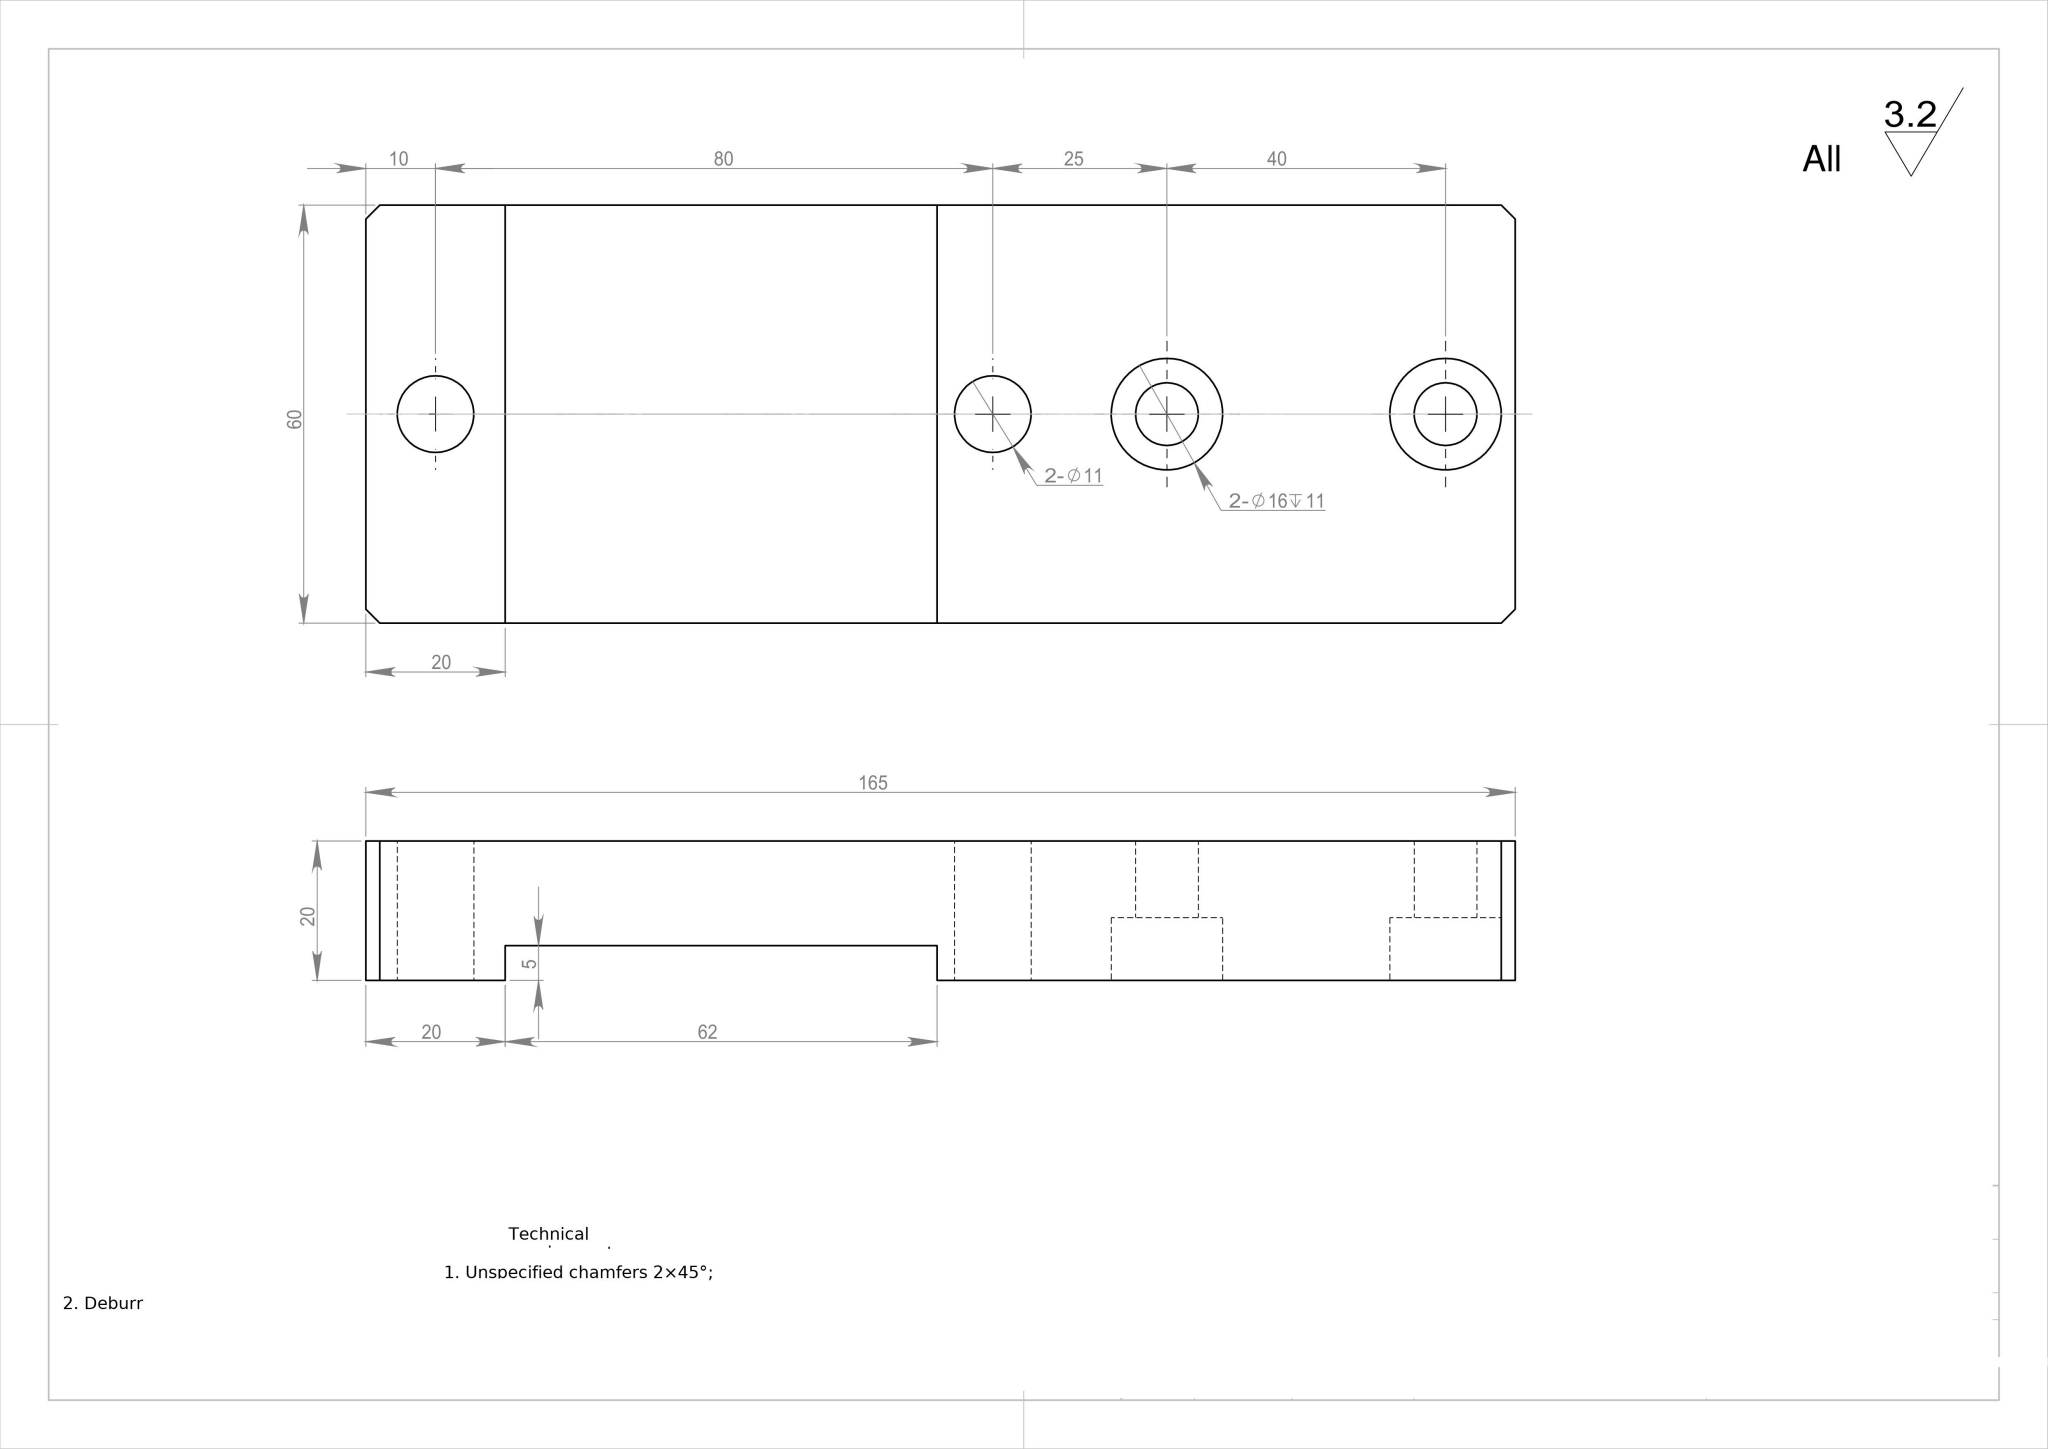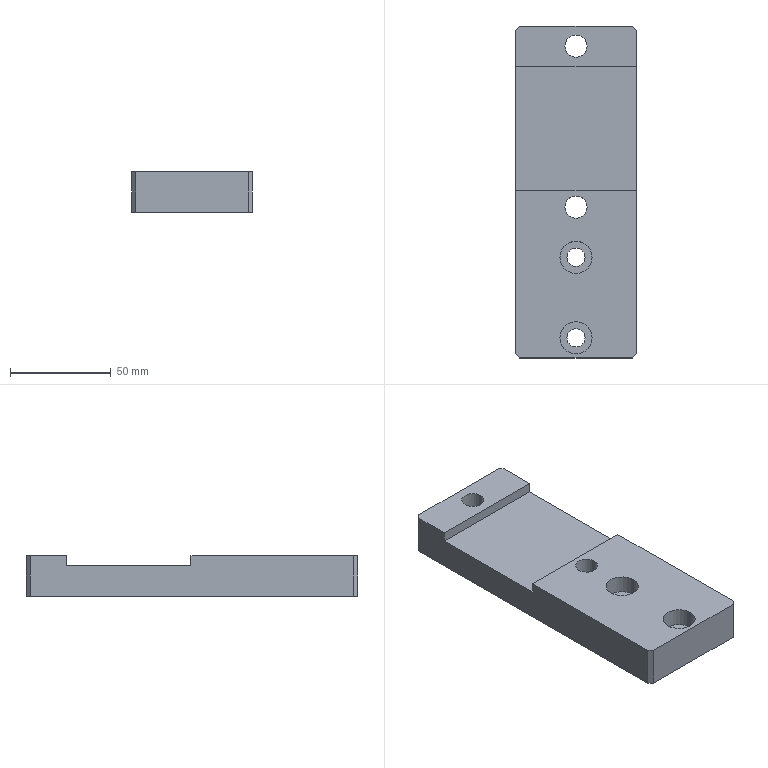Part | SolidWorks | mm | 1 solid | 28 faces | box 60 x 165 x 20 mm | volume 170420 mm3 | plane 16 | cylinder 12 | commonest cylinder face diameters 16 x4 9 x4 11 x4
build123d program:
from build123d import *

# Parameters (mm, degrees)
SKETCH1_W                                         = 60
SKETCH1_H                                         = 165
BOSS_EXTRUDE1_DEPTH                               = 20
SKETCH2_R                                         = 5.5
CUT_EXTRUDE1_DEPTH                                = 91.035
LPATTERN1_COUNT                                   = 2
LPATTERN1_PITCH                                   = 80
SKETCH3_W                                         = 60
SKETCH3_H                                         = 62
CUT_EXTRUDE2_DEPTH                                = 5
HOLE_SIZE_ACCORDING_TO_TYPE_1_OF_HEXA_D           = 9
HOLE_SIZE_ACCORDING_TO_TYPE_1_OF_HEXA_CBORE_D     = 16
HOLE_SIZE_ACCORDING_TO_TYPE_1_OF_HEXA_CBORE_DEPTH = 9
CHAMFER1_SIZE                                     = 2


with BuildPart() as part:
    # Sketch1 → Boss-Extrude1 (new body)
    with BuildSketch(Plane.XY):
        Rectangle(SKETCH1_W, SKETCH1_H)
    extrude(amount=BOSS_EXTRUDE1_DEPTH)

    # Sketch2 → Cut-Extrude1 (cut, through all)
    with BuildSketch(Plane(origin=(0, 0, 0), x_dir=(-1, 0, 0), z_dir=(0, 0, -1))):
        with Locations((0, 72.5)):
            Circle(SKETCH2_R)
    cut_extrude1 = extrude(amount=-CUT_EXTRUDE1_DEPTH, mode=Mode.SUBTRACT)

    # LPattern1: Cut-Extrude1 ×2
    with Locations(*[(0, -i * LPATTERN1_PITCH, 0) for i in range(1, LPATTERN1_COUNT)]):
        add(cut_extrude1, mode=Mode.SUBTRACT)

    # Sketch3 → Cut-Extrude2 (cut)
    with BuildSketch(Plane(origin=(0, 0, 20), x_dir=(-1, 0, 0), z_dir=(0, 0, -1))):
        with Locations((0, 31.5)):
            Rectangle(SKETCH3_W, SKETCH3_H)
    extrude(amount=CUT_EXTRUDE2_DEPTH, mode=Mode.SUBTRACT)

    # Hole Size _ according to_ Type 1 of Hexa (through all)
    with Locations(Plane.XY.offset(20)):
        with Locations((0, -32.5), (0, -72.5)):
            CounterBoreHole(HOLE_SIZE_ACCORDING_TO_TYPE_1_OF_HEXA_D / 2, HOLE_SIZE_ACCORDING_TO_TYPE_1_OF_HEXA_CBORE_D / 2, HOLE_SIZE_ACCORDING_TO_TYPE_1_OF_HEXA_CBORE_DEPTH)

    # Chamfer1
    chamfer1_edges = [part.edges().sort_by_distance(p)[0] for p in [
        (30, -82.5, 10),
        (-30, -82.5, 10),
        (-30, 82.5, 10),
        (30, 82.5, 10),
    ]]
    chamfer(chamfer1_edges, length=CHAMFER1_SIZE)


solid = part.part
STEP:
#1=CARTESIAN_POINT('',(-8.,-32.5,11.));
#2=VERTEX_POINT('',#1);
#3=CARTESIAN_POINT('',(8.,-32.5,11.));
#4=VERTEX_POINT('',#3);
#5=CARTESIAN_POINT('',(-0.,-32.5,11.));
#6=DIRECTION('',(0.,0.,1.));
#7=DIRECTION('',(1.,0.,0.));
#8=AXIS2_PLACEMENT_3D('',#5,#6,#7);
#9=CIRCLE('',#8,8.);
#10=EDGE_CURVE('',#2,#4,#9,.T.);
#11=ORIENTED_EDGE('',*,*,#10,.F.);
#12=CARTESIAN_POINT('',(-8.,-32.5,20.));
#13=VERTEX_POINT('',#12);
#14=CARTESIAN_POINT('',(-8.,-32.5,20.));
#15=DIRECTION('',(0.,0.,1.));
#16=VECTOR('',#15,1000.);
#17=LINE('',#14,#16);
#18=EDGE_CURVE('',#2,#13,#17,.T.);
#19=ORIENTED_EDGE('',*,*,#18,.T.);
#20=CARTESIAN_POINT('',(8.,-32.5,20.));
#21=VERTEX_POINT('',#20);
#22=CARTESIAN_POINT('',(-0.,-32.5,20.));
#23=DIRECTION('',(0.,0.,1.));
#24=DIRECTION('',(1.,0.,0.));
#25=AXIS2_PLACEMENT_3D('',#22,#23,#24);
#26=CIRCLE('',#25,8.);
#27=EDGE_CURVE('',#13,#21,#26,.T.);
#28=ORIENTED_EDGE('',*,*,#27,.T.);
#29=CARTESIAN_POINT('',(8.,-32.5,20.));
#30=DIRECTION('',(0.,0.,1.));
#31=VECTOR('',#30,1000.);
#32=LINE('',#29,#31);
#33=EDGE_CURVE('',#4,#21,#32,.T.);
#34=ORIENTED_EDGE('',*,*,#33,.F.);
#35=EDGE_LOOP('',(#11,#19,#28,#34));
#36=FACE_OUTER_BOUND('',#35,.T.);
#37=CARTESIAN_POINT('',(-0.,-32.5,20.));
#38=DIRECTION('',(0.,0.,1.));
#39=DIRECTION('',(1.,0.,0.));
#40=AXIS2_PLACEMENT_3D('',#37,#38,#39);
#41=CYLINDRICAL_SURFACE('',#40,8.);
#42=ADVANCED_FACE('',(#36),#41,.F.);
#43=CARTESIAN_POINT('',(-4.5,-32.5,0.));
#44=VERTEX_POINT('',#43);
#45=CARTESIAN_POINT('',(4.5,-32.5,0.));
#46=VERTEX_POINT('',#45);
#47=CARTESIAN_POINT('',(-0.,-32.5,0.));
#48=DIRECTION('',(0.,0.,1.));
#49=DIRECTION('',(1.,0.,0.));
#50=AXIS2_PLACEMENT_3D('',#47,#48,#49);
#51=CIRCLE('',#50,4.5);
#52=EDGE_CURVE('',#44,#46,#51,.T.);
#53=ORIENTED_EDGE('',*,*,#52,.F.);
#54=CARTESIAN_POINT('',(-4.5,-32.5,11.));
#55=VERTEX_POINT('',#54);
#56=CARTESIAN_POINT('',(-4.5,-32.5,20.));
#57=DIRECTION('',(0.,0.,1.));
#58=VECTOR('',#57,1000.);
#59=LINE('',#56,#58);
#60=EDGE_CURVE('',#44,#55,#59,.T.);
#61=ORIENTED_EDGE('',*,*,#60,.T.);
#62=CARTESIAN_POINT('',(4.5,-32.5,11.));
#63=VERTEX_POINT('',#62);
#64=CARTESIAN_POINT('',(-0.,-32.5,11.));
#65=DIRECTION('',(0.,0.,1.));
#66=DIRECTION('',(1.,0.,0.));
#67=AXIS2_PLACEMENT_3D('',#64,#65,#66);
#68=CIRCLE('',#67,4.5);
#69=EDGE_CURVE('',#55,#63,#68,.T.);
#70=ORIENTED_EDGE('',*,*,#69,.T.);
#71=CARTESIAN_POINT('',(4.5,-32.5,20.));
#72=DIRECTION('',(0.,0.,1.));
#73=VECTOR('',#72,1000.);
#74=LINE('',#71,#73);
#75=EDGE_CURVE('',#46,#63,#74,.T.);
#76=ORIENTED_EDGE('',*,*,#75,.F.);
#77=EDGE_LOOP('',(#53,#61,#70,#76));
#78=FACE_OUTER_BOUND('',#77,.T.);
#79=CARTESIAN_POINT('',(-0.,-32.5,20.));
#80=DIRECTION('',(0.,0.,1.));
#81=DIRECTION('',(1.,0.,0.));
#82=AXIS2_PLACEMENT_3D('',#79,#80,#81);
#83=CYLINDRICAL_SURFACE('',#82,4.5);
#84=ADVANCED_FACE('',(#78),#83,.F.);
#85=CARTESIAN_POINT('',(-8.,-72.5,11.));
#86=VERTEX_POINT('',#85);
#87=CARTESIAN_POINT('',(8.,-72.5,11.));
#88=VERTEX_POINT('',#87);
#89=CARTESIAN_POINT('',(-0.,-72.5,11.));
#90=DIRECTION('',(0.,0.,1.));
#91=DIRECTION('',(1.,0.,0.));
#92=AXIS2_PLACEMENT_3D('',#89,#90,#91);
#93=CIRCLE('',#92,8.);
#94=EDGE_CURVE('',#86,#88,#93,.T.);
#95=ORIENTED_EDGE('',*,*,#94,.F.);
#96=CARTESIAN_POINT('',(-8.,-72.5,20.));
#97=VERTEX_POINT('',#96);
#98=CARTESIAN_POINT('',(-8.,-72.5,20.));
#99=DIRECTION('',(0.,0.,1.));
#100=VECTOR('',#99,1000.);
#101=LINE('',#98,#100);
#102=EDGE_CURVE('',#86,#97,#101,.T.);
#103=ORIENTED_EDGE('',*,*,#102,.T.);
#104=CARTESIAN_POINT('',(8.,-72.5,20.));
#105=VERTEX_POINT('',#104);
#106=CARTESIAN_POINT('',(-0.,-72.5,20.));
#107=DIRECTION('',(0.,0.,1.));
#108=DIRECTION('',(1.,0.,0.));
#109=AXIS2_PLACEMENT_3D('',#106,#107,#108);
#110=CIRCLE('',#109,8.);
#111=EDGE_CURVE('',#97,#105,#110,.T.);
#112=ORIENTED_EDGE('',*,*,#111,.T.);
#113=CARTESIAN_POINT('',(8.,-72.5,20.));
#114=DIRECTION('',(0.,0.,1.));
#115=VECTOR('',#114,1000.);
#116=LINE('',#113,#115);
#117=EDGE_CURVE('',#88,#105,#116,.T.);
#118=ORIENTED_EDGE('',*,*,#117,.F.);
#119=EDGE_LOOP('',(#95,#103,#112,#118));
#120=FACE_OUTER_BOUND('',#119,.T.);
#121=CARTESIAN_POINT('',(-0.,-72.5,20.));
#122=DIRECTION('',(0.,0.,1.));
#123=DIRECTION('',(1.,0.,0.));
#124=AXIS2_PLACEMENT_3D('',#121,#122,#123);
#125=CYLINDRICAL_SURFACE('',#124,8.);
#126=ADVANCED_FACE('',(#120),#125,.F.);
#127=CARTESIAN_POINT('',(-4.5,-72.5,0.));
#128=VERTEX_POINT('',#127);
#129=CARTESIAN_POINT('',(4.5,-72.5,0.));
#130=VERTEX_POINT('',#129);
#131=CARTESIAN_POINT('',(-0.,-72.5,0.));
#132=DIRECTION('',(0.,0.,1.));
#133=DIRECTION('',(1.,0.,0.));
#134=AXIS2_PLACEMENT_3D('',#131,#132,#133);
#135=CIRCLE('',#134,4.5);
#136=EDGE_CURVE('',#128,#130,#135,.T.);
#137=ORIENTED_EDGE('',*,*,#136,.F.);
#138=CARTESIAN_POINT('',(-4.5,-72.5,11.));
#139=VERTEX_POINT('',#138);
#140=CARTESIAN_POINT('',(-4.5,-72.5,20.));
#141=DIRECTION('',(0.,0.,1.));
#142=VECTOR('',#141,1000.);
#143=LINE('',#140,#142);
#144=EDGE_CURVE('',#128,#139,#143,.T.);
#145=ORIENTED_EDGE('',*,*,#144,.T.);
#146=CARTESIAN_POINT('',(4.5,-72.5,11.));
#147=VERTEX_POINT('',#146);
#148=CARTESIAN_POINT('',(-0.,-72.5,11.));
#149=DIRECTION('',(0.,0.,1.));
#150=DIRECTION('',(1.,0.,0.));
#151=AXIS2_PLACEMENT_3D('',#148,#149,#150);
#152=CIRCLE('',#151,4.5);
#153=EDGE_CURVE('',#139,#147,#152,.T.);
#154=ORIENTED_EDGE('',*,*,#153,.T.);
#155=CARTESIAN_POINT('',(4.5,-72.5,20.));
#156=DIRECTION('',(0.,0.,1.));
#157=VECTOR('',#156,1000.);
#158=LINE('',#155,#157);
#159=EDGE_CURVE('',#130,#147,#158,.T.);
#160=ORIENTED_EDGE('',*,*,#159,.F.);
#161=EDGE_LOOP('',(#137,#145,#154,#160));
#162=FACE_OUTER_BOUND('',#161,.T.);
#163=CARTESIAN_POINT('',(-0.,-72.5,20.));
#164=DIRECTION('',(0.,0.,1.));
#165=DIRECTION('',(1.,0.,0.));
#166=AXIS2_PLACEMENT_3D('',#163,#164,#165);
#167=CYLINDRICAL_SURFACE('',#166,4.5);
#168=ADVANCED_FACE('',(#162),#167,.F.);
#169=CARTESIAN_POINT('',(5.5,-7.5,20.));
#170=VERTEX_POINT('',#169);
#171=CARTESIAN_POINT('',(-5.5,-7.5,20.));
#172=VERTEX_POINT('',#171);
#173=CARTESIAN_POINT('',(0.,-7.5,20.));
#174=DIRECTION('',(0.,0.,-1.));
#175=DIRECTION('',(-1.,0.,0.));
#176=AXIS2_PLACEMENT_3D('',#173,#174,#175);
#177=CIRCLE('',#176,5.5);
#178=EDGE_CURVE('',#170,#172,#177,.T.);
#179=ORIENTED_EDGE('',*,*,#178,.F.);
#180=CARTESIAN_POINT('',(5.5,-7.5,0.));
#181=VERTEX_POINT('',#180);
#182=CARTESIAN_POINT('',(5.5,-7.5,20.));
#183=DIRECTION('',(0.,0.,-1.));
#184=VECTOR('',#183,1000.);
#185=LINE('',#182,#184);
#186=EDGE_CURVE('',#170,#181,#185,.T.);
#187=ORIENTED_EDGE('',*,*,#186,.T.);
#188=CARTESIAN_POINT('',(-5.5,-7.5,0.));
#189=VERTEX_POINT('',#188);
#190=CARTESIAN_POINT('',(0.,-7.5,0.));
#191=DIRECTION('',(0.,0.,-1.));
#192=DIRECTION('',(-1.,0.,0.));
#193=AXIS2_PLACEMENT_3D('',#190,#191,#192);
#194=CIRCLE('',#193,5.5);
#195=EDGE_CURVE('',#181,#189,#194,.T.);
#196=ORIENTED_EDGE('',*,*,#195,.T.);
#197=CARTESIAN_POINT('',(-5.5,-7.5,20.));
#198=DIRECTION('',(0.,0.,-1.));
#199=VECTOR('',#198,1000.);
#200=LINE('',#197,#199);
#201=EDGE_CURVE('',#172,#189,#200,.T.);
#202=ORIENTED_EDGE('',*,*,#201,.F.);
#203=EDGE_LOOP('',(#179,#187,#196,#202));
#204=FACE_OUTER_BOUND('',#203,.T.);
#205=CARTESIAN_POINT('',(0.,-7.5,20.));
#206=DIRECTION('',(0.,0.,-1.));
#207=DIRECTION('',(-1.,0.,0.));
#208=AXIS2_PLACEMENT_3D('',#205,#206,#207);
#209=CYLINDRICAL_SURFACE('',#208,5.5);
#210=ADVANCED_FACE('',(#204),#209,.F.);
#211=CARTESIAN_POINT('',(5.5,72.5,20.));
#212=VERTEX_POINT('',#211);
#213=CARTESIAN_POINT('',(-5.5,72.5,20.));
#214=VERTEX_POINT('',#213);
#215=CARTESIAN_POINT('',(0.,72.5,20.));
#216=DIRECTION('',(0.,0.,-1.));
#217=DIRECTION('',(-1.,0.,0.));
#218=AXIS2_PLACEMENT_3D('',#215,#216,#217);
#219=CIRCLE('',#218,5.5);
#220=EDGE_CURVE('',#212,#214,#219,.T.);
#221=ORIENTED_EDGE('',*,*,#220,.F.);
#222=CARTESIAN_POINT('',(5.5,72.5,0.));
#223=VERTEX_POINT('',#222);
#224=CARTESIAN_POINT('',(5.5,72.5,20.));
#225=DIRECTION('',(0.,0.,-1.));
#226=VECTOR('',#225,1000.);
#227=LINE('',#224,#226);
#228=EDGE_CURVE('',#212,#223,#227,.T.);
#229=ORIENTED_EDGE('',*,*,#228,.T.);
#230=CARTESIAN_POINT('',(-5.5,72.5,0.));
#231=VERTEX_POINT('',#230);
#232=CARTESIAN_POINT('',(0.,72.5,0.));
#233=DIRECTION('',(0.,0.,-1.));
#234=DIRECTION('',(-1.,0.,0.));
#235=AXIS2_PLACEMENT_3D('',#232,#233,#234);
#236=CIRCLE('',#235,5.5);
#237=EDGE_CURVE('',#223,#231,#236,.T.);
#238=ORIENTED_EDGE('',*,*,#237,.T.);
#239=CARTESIAN_POINT('',(-5.5,72.5,20.));
#240=DIRECTION('',(0.,0.,-1.));
#241=VECTOR('',#240,1000.);
#242=LINE('',#239,#241);
#243=EDGE_CURVE('',#214,#231,#242,.T.);
#244=ORIENTED_EDGE('',*,*,#243,.F.);
#245=EDGE_LOOP('',(#221,#229,#238,#244));
#246=FACE_OUTER_BOUND('',#245,.T.);
#247=CARTESIAN_POINT('',(0.,72.5,20.));
#248=DIRECTION('',(0.,0.,-1.));
#249=DIRECTION('',(-1.,0.,0.));
#250=AXIS2_PLACEMENT_3D('',#247,#248,#249);
#251=CYLINDRICAL_SURFACE('',#250,5.5);
#252=ADVANCED_FACE('',(#246),#251,.F.);
#253=CARTESIAN_POINT('',(30.,-80.5,0.));
#254=VERTEX_POINT('',#253);
#255=CARTESIAN_POINT('',(30.,80.5,0.));
#256=VERTEX_POINT('',#255);
#257=CARTESIAN_POINT('',(30.,82.5,0.));
#258=DIRECTION('',(-0.,1.,0.));
#259=VECTOR('',#258,1000.);
#260=LINE('',#257,#259);
#261=EDGE_CURVE('',#254,#256,#260,.T.);
#262=ORIENTED_EDGE('',*,*,#261,.T.);
#263=CARTESIAN_POINT('',(30.,80.5,20.));
#264=VERTEX_POINT('',#263);
#265=CARTESIAN_POINT('',(30.,80.5,20.));
#266=DIRECTION('',(0.,0.,1.));
#267=VECTOR('',#266,1000.);
#268=LINE('',#265,#267);
#269=EDGE_CURVE('',#256,#264,#268,.T.);
#270=ORIENTED_EDGE('',*,*,#269,.T.);
#271=CARTESIAN_POINT('',(30.,62.5,20.));
#272=VERTEX_POINT('',#271);
#273=CARTESIAN_POINT('',(30.,82.5,20.));
#274=DIRECTION('',(-0.,1.,0.));
#275=VECTOR('',#274,1000.);
#276=LINE('',#273,#275);
#277=EDGE_CURVE('',#272,#264,#276,.T.);
#278=ORIENTED_EDGE('',*,*,#277,.F.);
#279=CARTESIAN_POINT('',(30.,62.5,15.));
#280=VERTEX_POINT('',#279);
#281=CARTESIAN_POINT('',(30.,62.5,15.));
#282=DIRECTION('',(0.,0.,1.));
#283=VECTOR('',#282,1000.);
#284=LINE('',#281,#283);
#285=EDGE_CURVE('',#280,#272,#284,.T.);
#286=ORIENTED_EDGE('',*,*,#285,.F.);
#287=CARTESIAN_POINT('',(30.,0.5,15.));
#288=VERTEX_POINT('',#287);
#289=CARTESIAN_POINT('',(30.,62.5,15.));
#290=DIRECTION('',(-0.,-1.,0.));
#291=VECTOR('',#290,1000.);
#292=LINE('',#289,#291);
#293=EDGE_CURVE('',#280,#288,#292,.T.);
#294=ORIENTED_EDGE('',*,*,#293,.T.);
#295=CARTESIAN_POINT('',(30.,0.5,20.));
#296=VERTEX_POINT('',#295);
#297=CARTESIAN_POINT('',(30.,0.5,15.));
#298=DIRECTION('',(0.,0.,1.));
#299=VECTOR('',#298,1000.);
#300=LINE('',#297,#299);
#301=EDGE_CURVE('',#288,#296,#300,.T.);
#302=ORIENTED_EDGE('',*,*,#301,.T.);
#303=CARTESIAN_POINT('',(30.,-80.5,20.));
#304=VERTEX_POINT('',#303);
#305=CARTESIAN_POINT('',(30.,82.5,20.));
#306=DIRECTION('',(-0.,1.,0.));
#307=VECTOR('',#306,1000.);
#308=LINE('',#305,#307);
#309=EDGE_CURVE('',#304,#296,#308,.T.);
#310=ORIENTED_EDGE('',*,*,#309,.F.);
#311=CARTESIAN_POINT('',(30.,-80.5,20.));
#312=DIRECTION('',(0.,0.,-1.));
#313=VECTOR('',#312,1000.);
#314=LINE('',#311,#313);
#315=EDGE_CURVE('',#304,#254,#314,.T.);
#316=ORIENTED_EDGE('',*,*,#315,.T.);
#317=EDGE_LOOP('',(#262,#270,#278,#286,#294,#302,#310,#316));
#318=FACE_OUTER_BOUND('',#317,.T.);
#319=CARTESIAN_POINT('',(30.,82.5,20.));
#320=DIRECTION('',(-1.,-0.,0.));
#321=DIRECTION('',(0.,-1.,0.));
#322=AXIS2_PLACEMENT_3D('',#319,#320,#321);
#323=PLANE('',#322);
#324=ADVANCED_FACE('',(#318),#323,.F.);
#325=CARTESIAN_POINT('',(-30.,80.5,20.));
#326=VERTEX_POINT('',#325);
#327=CARTESIAN_POINT('',(-30.,62.5,20.));
#328=VERTEX_POINT('',#327);
#329=CARTESIAN_POINT('',(-30.,82.5,20.));
#330=DIRECTION('',(0.,-1.,0.));
#331=VECTOR('',#330,1000.);
#332=LINE('',#329,#331);
#333=EDGE_CURVE('',#326,#328,#332,.T.);
#334=ORIENTED_EDGE('',*,*,#333,.F.);
#335=CARTESIAN_POINT('',(-30.,80.5,0.));
#336=VERTEX_POINT('',#335);
#337=CARTESIAN_POINT('',(-30.,80.5,20.));
#338=DIRECTION('',(0.,0.,-1.));
#339=VECTOR('',#338,1000.);
#340=LINE('',#337,#339);
#341=EDGE_CURVE('',#326,#336,#340,.T.);
#342=ORIENTED_EDGE('',*,*,#341,.T.);
#343=CARTESIAN_POINT('',(-30.,-80.5,0.));
#344=VERTEX_POINT('',#343);
#345=CARTESIAN_POINT('',(-30.,82.5,0.));
#346=DIRECTION('',(0.,-1.,0.));
#347=VECTOR('',#346,1000.);
#348=LINE('',#345,#347);
#349=EDGE_CURVE('',#336,#344,#348,.T.);
#350=ORIENTED_EDGE('',*,*,#349,.T.);
#351=CARTESIAN_POINT('',(-30.,-80.5,20.));
#352=VERTEX_POINT('',#351);
#353=CARTESIAN_POINT('',(-30.,-80.5,20.));
#354=DIRECTION('',(0.,0.,1.));
#355=VECTOR('',#354,1000.);
#356=LINE('',#353,#355);
#357=EDGE_CURVE('',#344,#352,#356,.T.);
#358=ORIENTED_EDGE('',*,*,#357,.T.);
#359=CARTESIAN_POINT('',(-30.,0.5,20.));
#360=VERTEX_POINT('',#359);
#361=CARTESIAN_POINT('',(-30.,82.5,20.));
#362=DIRECTION('',(0.,-1.,0.));
#363=VECTOR('',#362,1000.);
#364=LINE('',#361,#363);
#365=EDGE_CURVE('',#360,#352,#364,.T.);
#366=ORIENTED_EDGE('',*,*,#365,.F.);
#367=CARTESIAN_POINT('',(-30.,0.5,15.));
#368=VERTEX_POINT('',#367);
#369=CARTESIAN_POINT('',(-30.,0.5,15.));
#370=DIRECTION('',(0.,0.,1.));
#371=VECTOR('',#370,1000.);
#372=LINE('',#369,#371);
#373=EDGE_CURVE('',#368,#360,#372,.T.);
#374=ORIENTED_EDGE('',*,*,#373,.F.);
#375=CARTESIAN_POINT('',(-30.,62.5,15.));
#376=VERTEX_POINT('',#375);
#377=CARTESIAN_POINT('',(-30.,62.5,15.));
#378=DIRECTION('',(0.,1.,0.));
#379=VECTOR('',#378,1000.);
#380=LINE('',#377,#379);
#381=EDGE_CURVE('',#368,#376,#380,.T.);
#382=ORIENTED_EDGE('',*,*,#381,.T.);
#383=CARTESIAN_POINT('',(-30.,62.5,15.));
#384=DIRECTION('',(0.,0.,1.));
#385=VECTOR('',#384,1000.);
#386=LINE('',#383,#385);
#387=EDGE_CURVE('',#376,#328,#386,.T.);
#388=ORIENTED_EDGE('',*,*,#387,.T.);
#389=EDGE_LOOP('',(#334,#342,#350,#358,#366,#374,#382,#388));
#390=FACE_OUTER_BOUND('',#389,.T.);
#391=CARTESIAN_POINT('',(-30.,82.5,20.));
#392=DIRECTION('',(1.,0.,0.));
#393=DIRECTION('',(-0.,1.,0.));
#394=AXIS2_PLACEMENT_3D('',#391,#392,#393);
#395=PLANE('',#394);
#396=ADVANCED_FACE('',(#390),#395,.F.);
#397=CARTESIAN_POINT('',(-0.,-32.5,20.));
#398=DIRECTION('',(0.,0.,1.));
#399=DIRECTION('',(1.,0.,0.));
#400=AXIS2_PLACEMENT_3D('',#397,#398,#399);
#401=CIRCLE('',#400,8.);
#402=EDGE_CURVE('',#21,#13,#401,.T.);
#403=ORIENTED_EDGE('',*,*,#402,.F.);
#404=ORIENTED_EDGE('',*,*,#27,.F.);
#405=EDGE_LOOP('',(#403,#404));
#406=FACE_BOUND('',#405,.T.);
#407=CARTESIAN_POINT('',(-0.,-72.5,20.));
#408=DIRECTION('',(0.,0.,1.));
#409=DIRECTION('',(1.,0.,0.));
#410=AXIS2_PLACEMENT_3D('',#407,#408,#409);
#411=CIRCLE('',#410,8.);
#412=EDGE_CURVE('',#105,#97,#411,.T.);
#413=ORIENTED_EDGE('',*,*,#412,.F.);
#414=ORIENTED_EDGE('',*,*,#111,.F.);
#415=EDGE_LOOP('',(#413,#414));
#416=FACE_BOUND('',#415,.T.);
#417=CARTESIAN_POINT('',(0.,-7.5,20.));
#418=DIRECTION('',(0.,0.,-1.));
#419=DIRECTION('',(-1.,0.,0.));
#420=AXIS2_PLACEMENT_3D('',#417,#418,#419);
#421=CIRCLE('',#420,5.5);
#422=EDGE_CURVE('',#172,#170,#421,.T.);
#423=ORIENTED_EDGE('',*,*,#422,.T.);
#424=ORIENTED_EDGE('',*,*,#178,.T.);
#425=EDGE_LOOP('',(#423,#424));
#426=FACE_BOUND('',#425,.T.);
#427=CARTESIAN_POINT('',(-28.,-82.5,20.));
#428=VERTEX_POINT('',#427);
#429=CARTESIAN_POINT('',(28.,-82.5,20.));
#430=VERTEX_POINT('',#429);
#431=CARTESIAN_POINT('',(-30.,-82.5,20.));
#432=DIRECTION('',(1.,0.,0.));
#433=VECTOR('',#432,1000.);
#434=LINE('',#431,#433);
#435=EDGE_CURVE('',#428,#430,#434,.T.);
#436=ORIENTED_EDGE('',*,*,#435,.T.);
#437=CARTESIAN_POINT('',(55.25,-55.25,20.));
#438=DIRECTION('',(0.7071,0.7071,0.));
#439=VECTOR('',#438,1000.);
#440=LINE('',#437,#439);
#441=EDGE_CURVE('',#430,#304,#440,.T.);
#442=ORIENTED_EDGE('',*,*,#441,.T.);
#443=ORIENTED_EDGE('',*,*,#309,.T.);
#444=CARTESIAN_POINT('',(30.,0.5,20.));
#445=DIRECTION('',(-1.,0.,0.));
#446=VECTOR('',#445,1000.);
#447=LINE('',#444,#446);
#448=EDGE_CURVE('',#296,#360,#447,.T.);
#449=ORIENTED_EDGE('',*,*,#448,.T.);
#450=ORIENTED_EDGE('',*,*,#365,.T.);
#451=CARTESIAN_POINT('',(-55.25,-55.25,20.));
#452=DIRECTION('',(0.7071,-0.7071,0.));
#453=VECTOR('',#452,1000.);
#454=LINE('',#451,#453);
#455=EDGE_CURVE('',#352,#428,#454,.T.);
#456=ORIENTED_EDGE('',*,*,#455,.T.);
#457=EDGE_LOOP('',(#436,#442,#443,#449,#450,#456));
#458=FACE_OUTER_BOUND('',#457,.T.);
#459=CARTESIAN_POINT('',(0.,0.,20.));
#460=DIRECTION('',(0.,0.,1.));
#461=DIRECTION('',(1.,0.,0.));
#462=AXIS2_PLACEMENT_3D('',#459,#460,#461);
#463=PLANE('',#462);
#464=ADVANCED_FACE('',(#406,#416,#426,#458),#463,.T.);
#465=CARTESIAN_POINT('',(0.,72.5,20.));
#466=DIRECTION('',(0.,0.,-1.));
#467=DIRECTION('',(-1.,0.,0.));
#468=AXIS2_PLACEMENT_3D('',#465,#466,#467);
#469=CIRCLE('',#468,5.5);
#470=EDGE_CURVE('',#214,#212,#469,.T.);
#471=ORIENTED_EDGE('',*,*,#470,.T.);
#472=ORIENTED_EDGE('',*,*,#220,.T.);
#473=EDGE_LOOP('',(#471,#472));
#474=FACE_BOUND('',#473,.T.);
#475=CARTESIAN_POINT('',(28.,82.5,20.));
#476=VERTEX_POINT('',#475);
#477=CARTESIAN_POINT('',(-28.,82.5,20.));
#478=VERTEX_POINT('',#477);
#479=CARTESIAN_POINT('',(-30.,82.5,20.));
#480=DIRECTION('',(-1.,0.,0.));
#481=VECTOR('',#480,1000.);
#482=LINE('',#479,#481);
#483=EDGE_CURVE('',#476,#478,#482,.T.);
#484=ORIENTED_EDGE('',*,*,#483,.T.);
#485=CARTESIAN_POINT('',(-55.25,55.25,20.));
#486=DIRECTION('',(-0.7071,-0.7071,0.));
#487=VECTOR('',#486,1000.);
#488=LINE('',#485,#487);
#489=EDGE_CURVE('',#478,#326,#488,.T.);
#490=ORIENTED_EDGE('',*,*,#489,.T.);
#491=ORIENTED_EDGE('',*,*,#333,.T.);
#492=CARTESIAN_POINT('',(30.,62.5,20.));
#493=DIRECTION('',(1.,0.,0.));
#494=VECTOR('',#493,1000.);
#495=LINE('',#492,#494);
#496=EDGE_CURVE('',#328,#272,#495,.T.);
#497=ORIENTED_EDGE('',*,*,#496,.T.);
#498=ORIENTED_EDGE('',*,*,#277,.T.);
#499=CARTESIAN_POINT('',(55.25,55.25,20.));
#500=DIRECTION('',(-0.7071,0.7071,0.));
#501=VECTOR('',#500,1000.);
#502=LINE('',#499,#501);
#503=EDGE_CURVE('',#264,#476,#502,.T.);
#504=ORIENTED_EDGE('',*,*,#503,.T.);
#505=EDGE_LOOP('',(#484,#490,#491,#497,#498,#504));
#506=FACE_OUTER_BOUND('',#505,.T.);
#507=CARTESIAN_POINT('',(0.,0.,20.));
#508=DIRECTION('',(0.,0.,1.));
#509=DIRECTION('',(1.,0.,0.));
#510=AXIS2_PLACEMENT_3D('',#507,#508,#509);
#511=PLANE('',#510);
#512=ADVANCED_FACE('',(#474,#506),#511,.T.);
#513=CARTESIAN_POINT('',(28.,82.5,0.));
#514=VERTEX_POINT('',#513);
#515=CARTESIAN_POINT('',(-28.,82.5,0.));
#516=VERTEX_POINT('',#515);
#517=CARTESIAN_POINT('',(-30.,82.5,0.));
#518=DIRECTION('',(-1.,0.,0.));
#519=VECTOR('',#518,1000.);
#520=LINE('',#517,#519);
#521=EDGE_CURVE('',#514,#516,#520,.T.);
#522=ORIENTED_EDGE('',*,*,#521,.T.);
#523=CARTESIAN_POINT('',(-28.,82.5,20.));
#524=DIRECTION('',(0.,0.,1.));
#525=VECTOR('',#524,1000.);
#526=LINE('',#523,#525);
#527=EDGE_CURVE('',#516,#478,#526,.T.);
#528=ORIENTED_EDGE('',*,*,#527,.T.);
#529=ORIENTED_EDGE('',*,*,#483,.F.);
#530=CARTESIAN_POINT('',(28.,82.5,20.));
#531=DIRECTION('',(0.,0.,-1.));
#532=VECTOR('',#531,1000.);
#533=LINE('',#530,#532);
#534=EDGE_CURVE('',#476,#514,#533,.T.);
#535=ORIENTED_EDGE('',*,*,#534,.T.);
#536=EDGE_LOOP('',(#522,#528,#529,#535));
#537=FACE_OUTER_BOUND('',#536,.T.);
#538=CARTESIAN_POINT('',(-30.,82.5,20.));
#539=DIRECTION('',(0.,-1.,0.));
#540=DIRECTION('',(0.,0.,-1.));
#541=AXIS2_PLACEMENT_3D('',#538,#539,#540);
#542=PLANE('',#541);
#543=ADVANCED_FACE('',(#537),#542,.F.);
#544=CARTESIAN_POINT('',(-28.,-82.5,0.));
#545=VERTEX_POINT('',#544);
#546=CARTESIAN_POINT('',(28.,-82.5,0.));
#547=VERTEX_POINT('',#546);
#548=CARTESIAN_POINT('',(-30.,-82.5,0.));
#549=DIRECTION('',(1.,0.,0.));
#550=VECTOR('',#549,1000.);
#551=LINE('',#548,#550);
#552=EDGE_CURVE('',#545,#547,#551,.T.);
#553=ORIENTED_EDGE('',*,*,#552,.T.);
#554=CARTESIAN_POINT('',(28.,-82.5,20.));
#555=DIRECTION('',(0.,0.,1.));
#556=VECTOR('',#555,1000.);
#557=LINE('',#554,#556);
#558=EDGE_CURVE('',#547,#430,#557,.T.);
#559=ORIENTED_EDGE('',*,*,#558,.T.);
#560=ORIENTED_EDGE('',*,*,#435,.F.);
#561=CARTESIAN_POINT('',(-28.,-82.5,20.));
#562=DIRECTION('',(0.,0.,-1.));
#563=VECTOR('',#562,1000.);
#564=LINE('',#561,#563);
#565=EDGE_CURVE('',#428,#545,#564,.T.);
#566=ORIENTED_EDGE('',*,*,#565,.T.);
#567=EDGE_LOOP('',(#553,#559,#560,#566));
#568=FACE_OUTER_BOUND('',#567,.T.);
#569=CARTESIAN_POINT('',(-30.,-82.5,20.));
#570=DIRECTION('',(0.,1.,0.));
#571=DIRECTION('',(0.,0.,1.));
#572=AXIS2_PLACEMENT_3D('',#569,#570,#571);
#573=PLANE('',#572);
#574=ADVANCED_FACE('',(#568),#573,.F.);
#575=CARTESIAN_POINT('',(-0.,-32.5,0.));
#576=DIRECTION('',(0.,0.,1.));
#577=DIRECTION('',(1.,0.,0.));
#578=AXIS2_PLACEMENT_3D('',#575,#576,#577);
#579=CIRCLE('',#578,4.5);
#580=EDGE_CURVE('',#46,#44,#579,.T.);
#581=ORIENTED_EDGE('',*,*,#580,.T.);
#582=ORIENTED_EDGE('',*,*,#52,.T.);
#583=EDGE_LOOP('',(#581,#582));
#584=FACE_BOUND('',#583,.T.);
#585=CARTESIAN_POINT('',(-0.,-72.5,0.));
#586=DIRECTION('',(0.,0.,1.));
#587=DIRECTION('',(1.,0.,0.));
#588=AXIS2_PLACEMENT_3D('',#585,#586,#587);
#589=CIRCLE('',#588,4.5);
#590=EDGE_CURVE('',#130,#128,#589,.T.);
#591=ORIENTED_EDGE('',*,*,#590,.T.);
#592=ORIENTED_EDGE('',*,*,#136,.T.);
#593=EDGE_LOOP('',(#591,#592));
#594=FACE_BOUND('',#593,.T.);
#595=CARTESIAN_POINT('',(0.,-7.5,0.));
#596=DIRECTION('',(0.,0.,-1.));
#597=DIRECTION('',(-1.,0.,0.));
#598=AXIS2_PLACEMENT_3D('',#595,#596,#597);
#599=CIRCLE('',#598,5.5);
#600=EDGE_CURVE('',#189,#181,#599,.T.);
#601=ORIENTED_EDGE('',*,*,#600,.F.);
#602=ORIENTED_EDGE('',*,*,#195,.F.);
#603=EDGE_LOOP('',(#601,#602));
#604=FACE_BOUND('',#603,.T.);
#605=CARTESIAN_POINT('',(0.,72.5,0.));
#606=DIRECTION('',(0.,0.,-1.));
#607=DIRECTION('',(-1.,0.,0.));
#608=AXIS2_PLACEMENT_3D('',#605,#606,#607);
#609=CIRCLE('',#608,5.5);
#610=EDGE_CURVE('',#231,#223,#609,.T.);
#611=ORIENTED_EDGE('',*,*,#610,.F.);
#612=ORIENTED_EDGE('',*,*,#237,.F.);
#613=EDGE_LOOP('',(#611,#612));
#614=FACE_BOUND('',#613,.T.);
#615=ORIENTED_EDGE('',*,*,#349,.F.);
#616=CARTESIAN_POINT('',(-30.,80.5,0.));
#617=DIRECTION('',(0.7071,0.7071,0.));
#618=VECTOR('',#617,1000.);
#619=LINE('',#616,#618);
#620=EDGE_CURVE('',#336,#516,#619,.T.);
#621=ORIENTED_EDGE('',*,*,#620,.T.);
#622=ORIENTED_EDGE('',*,*,#521,.F.);
#623=CARTESIAN_POINT('',(28.,82.5,0.));
#624=DIRECTION('',(0.7071,-0.7071,0.));
#625=VECTOR('',#624,1000.);
#626=LINE('',#623,#625);
#627=EDGE_CURVE('',#514,#256,#626,.T.);
#628=ORIENTED_EDGE('',*,*,#627,.T.);
#629=ORIENTED_EDGE('',*,*,#261,.F.);
#630=CARTESIAN_POINT('',(30.,-80.5,0.));
#631=DIRECTION('',(-0.7071,-0.7071,0.));
#632=VECTOR('',#631,1000.);
#633=LINE('',#630,#632);
#634=EDGE_CURVE('',#254,#547,#633,.T.);
#635=ORIENTED_EDGE('',*,*,#634,.T.);
#636=ORIENTED_EDGE('',*,*,#552,.F.);
#637=CARTESIAN_POINT('',(-28.,-82.5,0.));
#638=DIRECTION('',(-0.7071,0.7071,0.));
#639=VECTOR('',#638,1000.);
#640=LINE('',#637,#639);
#641=EDGE_CURVE('',#545,#344,#640,.T.);
#642=ORIENTED_EDGE('',*,*,#641,.T.);
#643=EDGE_LOOP('',(#615,#621,#622,#628,#629,#635,#636,#642));
#644=FACE_OUTER_BOUND('',#643,.T.);
#645=CARTESIAN_POINT('',(0.,0.,0.));
#646=DIRECTION('',(0.,0.,1.));
#647=DIRECTION('',(1.,0.,0.));
#648=AXIS2_PLACEMENT_3D('',#645,#646,#647);
#649=PLANE('',#648);
#650=ADVANCED_FACE('',(#584,#594,#604,#614,#644),#649,.F.);
#651=ORIENTED_EDGE('',*,*,#228,.F.);
#652=ORIENTED_EDGE('',*,*,#470,.F.);
#653=ORIENTED_EDGE('',*,*,#243,.T.);
#654=ORIENTED_EDGE('',*,*,#610,.T.);
#655=EDGE_LOOP('',(#651,#652,#653,#654));
#656=FACE_OUTER_BOUND('',#655,.T.);
#657=CARTESIAN_POINT('',(0.,72.5,20.));
#658=DIRECTION('',(0.,0.,-1.));
#659=DIRECTION('',(-1.,0.,0.));
#660=AXIS2_PLACEMENT_3D('',#657,#658,#659);
#661=CYLINDRICAL_SURFACE('',#660,5.5);
#662=ADVANCED_FACE('',(#656),#661,.F.);
#663=ORIENTED_EDGE('',*,*,#186,.F.);
#664=ORIENTED_EDGE('',*,*,#422,.F.);
#665=ORIENTED_EDGE('',*,*,#201,.T.);
#666=ORIENTED_EDGE('',*,*,#600,.T.);
#667=EDGE_LOOP('',(#663,#664,#665,#666));
#668=FACE_OUTER_BOUND('',#667,.T.);
#669=CARTESIAN_POINT('',(0.,-7.5,20.));
#670=DIRECTION('',(0.,0.,-1.));
#671=DIRECTION('',(-1.,0.,0.));
#672=AXIS2_PLACEMENT_3D('',#669,#670,#671);
#673=CYLINDRICAL_SURFACE('',#672,5.5);
#674=ADVANCED_FACE('',(#668),#673,.F.);
#675=ORIENTED_EDGE('',*,*,#448,.F.);
#676=ORIENTED_EDGE('',*,*,#301,.F.);
#677=CARTESIAN_POINT('',(30.,0.5,15.));
#678=DIRECTION('',(-1.,0.,0.));
#679=VECTOR('',#678,1000.);
#680=LINE('',#677,#679);
#681=EDGE_CURVE('',#288,#368,#680,.T.);
#682=ORIENTED_EDGE('',*,*,#681,.T.);
#683=ORIENTED_EDGE('',*,*,#373,.T.);
#684=EDGE_LOOP('',(#675,#676,#682,#683));
#685=FACE_OUTER_BOUND('',#684,.T.);
#686=CARTESIAN_POINT('',(30.,0.5,15.));
#687=DIRECTION('',(0.,1.,0.));
#688=DIRECTION('',(0.,0.,1.));
#689=AXIS2_PLACEMENT_3D('',#686,#687,#688);
#690=PLANE('',#689);
#691=ADVANCED_FACE('',(#685),#690,.T.);
#692=ORIENTED_EDGE('',*,*,#496,.F.);
#693=ORIENTED_EDGE('',*,*,#387,.F.);
#694=CARTESIAN_POINT('',(30.,62.5,15.));
#695=DIRECTION('',(1.,0.,0.));
#696=VECTOR('',#695,1000.);
#697=LINE('',#694,#696);
#698=EDGE_CURVE('',#376,#280,#697,.T.);
#699=ORIENTED_EDGE('',*,*,#698,.T.);
#700=ORIENTED_EDGE('',*,*,#285,.T.);
#701=EDGE_LOOP('',(#692,#693,#699,#700));
#702=FACE_OUTER_BOUND('',#701,.T.);
#703=CARTESIAN_POINT('',(30.,62.5,15.));
#704=DIRECTION('',(0.,-1.,0.));
#705=DIRECTION('',(1.,0.,0.));
#706=AXIS2_PLACEMENT_3D('',#703,#704,#705);
#707=PLANE('',#706);
#708=ADVANCED_FACE('',(#702),#707,.T.);
#709=ORIENTED_EDGE('',*,*,#293,.F.);
#710=ORIENTED_EDGE('',*,*,#698,.F.);
#711=ORIENTED_EDGE('',*,*,#381,.F.);
#712=ORIENTED_EDGE('',*,*,#681,.F.);
#713=EDGE_LOOP('',(#709,#710,#711,#712));
#714=FACE_OUTER_BOUND('',#713,.T.);
#715=CARTESIAN_POINT('',(0.,0.,15.));
#716=DIRECTION('',(0.,0.,-1.));
#717=DIRECTION('',(-1.,0.,0.));
#718=AXIS2_PLACEMENT_3D('',#715,#716,#717);
#719=PLANE('',#718);
#720=ADVANCED_FACE('',(#714),#719,.F.);
#721=ORIENTED_EDGE('',*,*,#144,.F.);
#722=ORIENTED_EDGE('',*,*,#590,.F.);
#723=ORIENTED_EDGE('',*,*,#159,.T.);
#724=CARTESIAN_POINT('',(-0.,-72.5,11.));
#725=DIRECTION('',(0.,0.,1.));
#726=DIRECTION('',(1.,0.,0.));
#727=AXIS2_PLACEMENT_3D('',#724,#725,#726);
#728=CIRCLE('',#727,4.5);
#729=EDGE_CURVE('',#147,#139,#728,.T.);
#730=ORIENTED_EDGE('',*,*,#729,.T.);
#731=EDGE_LOOP('',(#721,#722,#723,#730));
#732=FACE_OUTER_BOUND('',#731,.T.);
#733=CARTESIAN_POINT('',(-0.,-72.5,20.));
#734=DIRECTION('',(0.,0.,1.));
#735=DIRECTION('',(1.,0.,0.));
#736=AXIS2_PLACEMENT_3D('',#733,#734,#735);
#737=CYLINDRICAL_SURFACE('',#736,4.5);
#738=ADVANCED_FACE('',(#732),#737,.F.);
#739=ORIENTED_EDGE('',*,*,#729,.F.);
#740=ORIENTED_EDGE('',*,*,#153,.F.);
#741=EDGE_LOOP('',(#739,#740));
#742=FACE_BOUND('',#741,.T.);
#743=CARTESIAN_POINT('',(-0.,-72.5,11.));
#744=DIRECTION('',(0.,0.,1.));
#745=DIRECTION('',(1.,0.,0.));
#746=AXIS2_PLACEMENT_3D('',#743,#744,#745);
#747=CIRCLE('',#746,8.);
#748=EDGE_CURVE('',#88,#86,#747,.T.);
#749=ORIENTED_EDGE('',*,*,#748,.T.);
#750=ORIENTED_EDGE('',*,*,#94,.T.);
#751=EDGE_LOOP('',(#749,#750));
#752=FACE_OUTER_BOUND('',#751,.T.);
#753=CARTESIAN_POINT('',(4.5,-72.5,11.));
#754=DIRECTION('',(0.,0.,-1.));
#755=DIRECTION('',(-1.,0.,0.));
#756=AXIS2_PLACEMENT_3D('',#753,#754,#755);
#757=PLANE('',#756);
#758=ADVANCED_FACE('',(#742,#752),#757,.F.);
#759=ORIENTED_EDGE('',*,*,#102,.F.);
#760=ORIENTED_EDGE('',*,*,#748,.F.);
#761=ORIENTED_EDGE('',*,*,#117,.T.);
#762=ORIENTED_EDGE('',*,*,#412,.T.);
#763=EDGE_LOOP('',(#759,#760,#761,#762));
#764=FACE_OUTER_BOUND('',#763,.T.);
#765=CARTESIAN_POINT('',(-0.,-72.5,20.));
#766=DIRECTION('',(0.,0.,1.));
#767=DIRECTION('',(1.,0.,0.));
#768=AXIS2_PLACEMENT_3D('',#765,#766,#767);
#769=CYLINDRICAL_SURFACE('',#768,8.);
#770=ADVANCED_FACE('',(#764),#769,.F.);
#771=ORIENTED_EDGE('',*,*,#60,.F.);
#772=ORIENTED_EDGE('',*,*,#580,.F.);
#773=ORIENTED_EDGE('',*,*,#75,.T.);
#774=CARTESIAN_POINT('',(-0.,-32.5,11.));
#775=DIRECTION('',(0.,0.,1.));
#776=DIRECTION('',(1.,0.,0.));
#777=AXIS2_PLACEMENT_3D('',#774,#775,#776);
#778=CIRCLE('',#777,4.5);
#779=EDGE_CURVE('',#63,#55,#778,.T.);
#780=ORIENTED_EDGE('',*,*,#779,.T.);
#781=EDGE_LOOP('',(#771,#772,#773,#780));
#782=FACE_OUTER_BOUND('',#781,.T.);
#783=CARTESIAN_POINT('',(-0.,-32.5,20.));
#784=DIRECTION('',(0.,0.,1.));
#785=DIRECTION('',(1.,0.,0.));
#786=AXIS2_PLACEMENT_3D('',#783,#784,#785);
#787=CYLINDRICAL_SURFACE('',#786,4.5);
#788=ADVANCED_FACE('',(#782),#787,.F.);
#789=ORIENTED_EDGE('',*,*,#779,.F.);
#790=ORIENTED_EDGE('',*,*,#69,.F.);
#791=EDGE_LOOP('',(#789,#790));
#792=FACE_BOUND('',#791,.T.);
#793=CARTESIAN_POINT('',(-0.,-32.5,11.));
#794=DIRECTION('',(0.,0.,1.));
#795=DIRECTION('',(1.,0.,0.));
#796=AXIS2_PLACEMENT_3D('',#793,#794,#795);
#797=CIRCLE('',#796,8.);
#798=EDGE_CURVE('',#4,#2,#797,.T.);
#799=ORIENTED_EDGE('',*,*,#798,.T.);
#800=ORIENTED_EDGE('',*,*,#10,.T.);
#801=EDGE_LOOP('',(#799,#800));
#802=FACE_OUTER_BOUND('',#801,.T.);
#803=CARTESIAN_POINT('',(4.5,-32.5,11.));
#804=DIRECTION('',(0.,0.,-1.));
#805=DIRECTION('',(-1.,0.,0.));
#806=AXIS2_PLACEMENT_3D('',#803,#804,#805);
#807=PLANE('',#806);
#808=ADVANCED_FACE('',(#792,#802),#807,.F.);
#809=ORIENTED_EDGE('',*,*,#18,.F.);
#810=ORIENTED_EDGE('',*,*,#798,.F.);
#811=ORIENTED_EDGE('',*,*,#33,.T.);
#812=ORIENTED_EDGE('',*,*,#402,.T.);
#813=EDGE_LOOP('',(#809,#810,#811,#812));
#814=FACE_OUTER_BOUND('',#813,.T.);
#815=CARTESIAN_POINT('',(-0.,-32.5,20.));
#816=DIRECTION('',(0.,0.,1.));
#817=DIRECTION('',(1.,0.,0.));
#818=AXIS2_PLACEMENT_3D('',#815,#816,#817);
#819=CYLINDRICAL_SURFACE('',#818,8.);
#820=ADVANCED_FACE('',(#814),#819,.F.);
#821=ORIENTED_EDGE('',*,*,#489,.F.);
#822=ORIENTED_EDGE('',*,*,#527,.F.);
#823=ORIENTED_EDGE('',*,*,#620,.F.);
#824=ORIENTED_EDGE('',*,*,#341,.F.);
#825=EDGE_LOOP('',(#821,#822,#823,#824));
#826=FACE_OUTER_BOUND('',#825,.T.);
#827=CARTESIAN_POINT('',(-30.,80.5,20.));
#828=DIRECTION('',(0.7071,-0.7071,0.));
#829=DIRECTION('',(0.,0.,-1.));
#830=AXIS2_PLACEMENT_3D('',#827,#828,#829);
#831=PLANE('',#830);
#832=ADVANCED_FACE('',(#826),#831,.F.);
#833=ORIENTED_EDGE('',*,*,#503,.F.);
#834=ORIENTED_EDGE('',*,*,#269,.F.);
#835=ORIENTED_EDGE('',*,*,#627,.F.);
#836=ORIENTED_EDGE('',*,*,#534,.F.);
#837=EDGE_LOOP('',(#833,#834,#835,#836));
#838=FACE_OUTER_BOUND('',#837,.T.);
#839=CARTESIAN_POINT('',(28.,82.5,20.));
#840=DIRECTION('',(-0.7071,-0.7071,0.));
#841=DIRECTION('',(0.,0.,-1.));
#842=AXIS2_PLACEMENT_3D('',#839,#840,#841);
#843=PLANE('',#842);
#844=ADVANCED_FACE('',(#838),#843,.F.);
#845=ORIENTED_EDGE('',*,*,#441,.F.);
#846=ORIENTED_EDGE('',*,*,#558,.F.);
#847=ORIENTED_EDGE('',*,*,#634,.F.);
#848=ORIENTED_EDGE('',*,*,#315,.F.);
#849=EDGE_LOOP('',(#845,#846,#847,#848));
#850=FACE_OUTER_BOUND('',#849,.T.);
#851=CARTESIAN_POINT('',(30.,-80.5,20.));
#852=DIRECTION('',(-0.7071,0.7071,0.));
#853=DIRECTION('',(0.,0.,-1.));
#854=AXIS2_PLACEMENT_3D('',#851,#852,#853);
#855=PLANE('',#854);
#856=ADVANCED_FACE('',(#850),#855,.F.);
#857=ORIENTED_EDGE('',*,*,#455,.F.);
#858=ORIENTED_EDGE('',*,*,#357,.F.);
#859=ORIENTED_EDGE('',*,*,#641,.F.);
#860=ORIENTED_EDGE('',*,*,#565,.F.);
#861=EDGE_LOOP('',(#857,#858,#859,#860));
#862=FACE_OUTER_BOUND('',#861,.T.);
#863=CARTESIAN_POINT('',(-28.,-82.5,20.));
#864=DIRECTION('',(0.7071,0.7071,0.));
#865=DIRECTION('',(0.,0.,-1.));
#866=AXIS2_PLACEMENT_3D('',#863,#864,#865);
#867=PLANE('',#866);
#868=ADVANCED_FACE('',(#862),#867,.F.);
#869=CLOSED_SHELL('',(#42,#84,#126,#168,#210,#252,#324,#396,#464,#512,#543,#574,#650,#662,#674,#691,#708,#720,#738,#758,#770,#788,#808,#820,#832,#844,#856,#868));
#870=MANIFOLD_SOLID_BREP('',#869);
#871=CARTESIAN_POINT('',(0.,0.,0.));
#872=DIRECTION('',(0.,0.,1.));
#873=DIRECTION('',(1.,0.,0.));
#874=AXIS2_PLACEMENT_3D('',#871,#872,#873);
#875=(LENGTH_UNIT()NAMED_UNIT(*)SI_UNIT(.MILLI.,.METRE.));
#876=UNCERTAINTY_MEASURE_WITH_UNIT(LENGTH_MEASURE(0.00001),#875,'','');
#877=(NAMED_UNIT(*)PLANE_ANGLE_UNIT()SI_UNIT($,.RADIAN.));
#878=(NAMED_UNIT(*)SI_UNIT($,.STERADIAN.)SOLID_ANGLE_UNIT());
#879=(GEOMETRIC_REPRESENTATION_CONTEXT(3)GLOBAL_UNCERTAINTY_ASSIGNED_CONTEXT((#876))GLOBAL_UNIT_ASSIGNED_CONTEXT((#875,#877,#878))REPRESENTATION_CONTEXT('',''));
#880=ADVANCED_BREP_SHAPE_REPRESENTATION('',(#870,#874),#879);